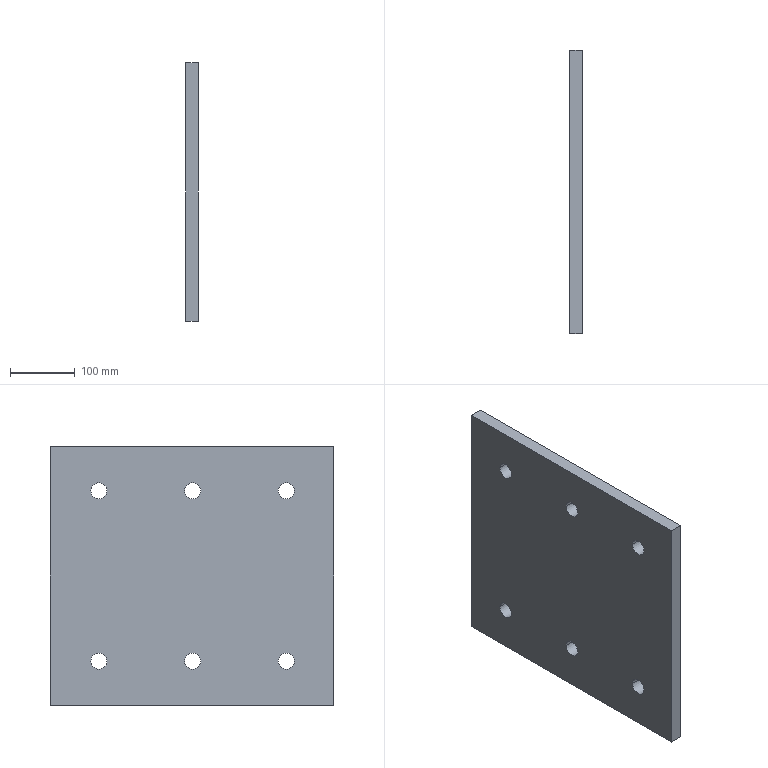Component | SolidWorks | ConnectingPlate-1 | 1 solid | 18 faces | box 20 x 438 x 400 mm | volume 3445095 mm3 | cylinder 12 | plane 6 | commonest cylinder face diameters 25 x12 | material Plain Carbon Steel
STEP:
#1=COLOUR_RGB('',0.7922,0.8196,0.9333);
#2=FILL_AREA_STYLE_COLOUR('',#1);
#3=FILL_AREA_STYLE('',(#2));
#4=SURFACE_STYLE_FILL_AREA(#3);
#5=SURFACE_SIDE_STYLE('',(#4));
#6=SURFACE_STYLE_USAGE(.BOTH.,#5);
#7=PRESENTATION_STYLE_ASSIGNMENT((#6));
#8=CARTESIAN_POINT('',(654.919,112.492,67.853));
#9=VERTEX_POINT('',#8);
#10=CARTESIAN_POINT('',(654.919,111.508,67.853));
#11=VERTEX_POINT('',#10);
#12=CARTESIAN_POINT('',(654.919,112.,67.853));
#13=DIRECTION('',(1.,-0.,-0.));
#14=DIRECTION('',(0.,1.,0.));
#15=AXIS2_PLACEMENT_3D('',#12,#13,#14);
#16=CIRCLE('',#15,0.4921);
#17=EDGE_CURVE('',#9,#11,#16,.T.);
#18=ORIENTED_EDGE('',*,*,#17,.F.);
#19=CARTESIAN_POINT('',(655.706,112.492,67.853));
#20=VERTEX_POINT('',#19);
#21=CARTESIAN_POINT('',(654.919,112.492,67.853));
#22=DIRECTION('',(1.,-0.,-0.));
#23=VECTOR('',#22,39.37);
#24=LINE('',#21,#23);
#25=EDGE_CURVE('',#9,#20,#24,.T.);
#26=ORIENTED_EDGE('',*,*,#25,.T.);
#27=CARTESIAN_POINT('',(655.706,111.508,67.853));
#28=VERTEX_POINT('',#27);
#29=CARTESIAN_POINT('',(655.706,112.,67.853));
#30=DIRECTION('',(1.,-0.,-0.));
#31=DIRECTION('',(0.,1.,0.));
#32=AXIS2_PLACEMENT_3D('',#29,#30,#31);
#33=CIRCLE('',#32,0.4921);
#34=EDGE_CURVE('',#20,#28,#33,.T.);
#35=ORIENTED_EDGE('',*,*,#34,.T.);
#36=CARTESIAN_POINT('',(654.919,111.508,67.853));
#37=DIRECTION('',(1.,-0.,-0.));
#38=VECTOR('',#37,39.37);
#39=LINE('',#36,#38);
#40=EDGE_CURVE('',#11,#28,#39,.T.);
#41=ORIENTED_EDGE('',*,*,#40,.F.);
#42=EDGE_LOOP('',(#18,#26,#35,#41));
#43=FACE_OUTER_BOUND('',#42,.T.);
#44=CARTESIAN_POINT('',(654.919,112.,67.853));
#45=DIRECTION('',(1.,-0.,-0.));
#46=DIRECTION('',(0.,-1.,0.));
#47=AXIS2_PLACEMENT_3D('',#44,#45,#46);
#48=CYLINDRICAL_SURFACE('',#47,0.4921);
#49=ADVANCED_FACE('',(#43),#48,.F.);
#50=CARTESIAN_POINT('',(654.919,106.784,67.853));
#51=VERTEX_POINT('',#50);
#52=CARTESIAN_POINT('',(654.919,105.799,67.853));
#53=VERTEX_POINT('',#52);
#54=CARTESIAN_POINT('',(654.919,106.291,67.853));
#55=DIRECTION('',(1.,-0.,-0.));
#56=DIRECTION('',(0.,1.,0.));
#57=AXIS2_PLACEMENT_3D('',#54,#55,#56);
#58=CIRCLE('',#57,0.4921);
#59=EDGE_CURVE('',#51,#53,#58,.T.);
#60=ORIENTED_EDGE('',*,*,#59,.F.);
#61=CARTESIAN_POINT('',(655.706,106.784,67.853));
#62=VERTEX_POINT('',#61);
#63=CARTESIAN_POINT('',(654.919,106.784,67.853));
#64=DIRECTION('',(1.,-0.,-0.));
#65=VECTOR('',#64,39.37);
#66=LINE('',#63,#65);
#67=EDGE_CURVE('',#51,#62,#66,.T.);
#68=ORIENTED_EDGE('',*,*,#67,.T.);
#69=CARTESIAN_POINT('',(655.706,105.799,67.853));
#70=VERTEX_POINT('',#69);
#71=CARTESIAN_POINT('',(655.706,106.291,67.853));
#72=DIRECTION('',(1.,-0.,-0.));
#73=DIRECTION('',(0.,1.,0.));
#74=AXIS2_PLACEMENT_3D('',#71,#72,#73);
#75=CIRCLE('',#74,0.4921);
#76=EDGE_CURVE('',#62,#70,#75,.T.);
#77=ORIENTED_EDGE('',*,*,#76,.T.);
#78=CARTESIAN_POINT('',(654.919,105.799,67.853));
#79=DIRECTION('',(1.,-0.,-0.));
#80=VECTOR('',#79,39.37);
#81=LINE('',#78,#80);
#82=EDGE_CURVE('',#53,#70,#81,.T.);
#83=ORIENTED_EDGE('',*,*,#82,.F.);
#84=EDGE_LOOP('',(#60,#68,#77,#83));
#85=FACE_OUTER_BOUND('',#84,.T.);
#86=CARTESIAN_POINT('',(654.919,106.291,67.853));
#87=DIRECTION('',(1.,-0.,-0.));
#88=DIRECTION('',(0.,-1.,0.));
#89=AXIS2_PLACEMENT_3D('',#86,#87,#88);
#90=CYLINDRICAL_SURFACE('',#89,0.4921);
#91=ADVANCED_FACE('',(#85),#90,.F.);
#92=CARTESIAN_POINT('',(654.919,101.075,67.853));
#93=VERTEX_POINT('',#92);
#94=CARTESIAN_POINT('',(654.919,100.091,67.853));
#95=VERTEX_POINT('',#94);
#96=CARTESIAN_POINT('',(654.919,100.583,67.853));
#97=DIRECTION('',(1.,-0.,-0.));
#98=DIRECTION('',(0.,1.,0.));
#99=AXIS2_PLACEMENT_3D('',#96,#97,#98);
#100=CIRCLE('',#99,0.4921);
#101=EDGE_CURVE('',#93,#95,#100,.T.);
#102=ORIENTED_EDGE('',*,*,#101,.F.);
#103=CARTESIAN_POINT('',(655.706,101.075,67.853));
#104=VERTEX_POINT('',#103);
#105=CARTESIAN_POINT('',(654.919,101.075,67.853));
#106=DIRECTION('',(1.,-0.,-0.));
#107=VECTOR('',#106,39.37);
#108=LINE('',#105,#107);
#109=EDGE_CURVE('',#93,#104,#108,.T.);
#110=ORIENTED_EDGE('',*,*,#109,.T.);
#111=CARTESIAN_POINT('',(655.706,100.091,67.853));
#112=VERTEX_POINT('',#111);
#113=CARTESIAN_POINT('',(655.706,100.583,67.853));
#114=DIRECTION('',(1.,-0.,-0.));
#115=DIRECTION('',(0.,1.,0.));
#116=AXIS2_PLACEMENT_3D('',#113,#114,#115);
#117=CIRCLE('',#116,0.4921);
#118=EDGE_CURVE('',#104,#112,#117,.T.);
#119=ORIENTED_EDGE('',*,*,#118,.T.);
#120=CARTESIAN_POINT('',(654.919,100.091,67.853));
#121=DIRECTION('',(1.,-0.,-0.));
#122=VECTOR('',#121,39.37);
#123=LINE('',#120,#122);
#124=EDGE_CURVE('',#95,#112,#123,.T.);
#125=ORIENTED_EDGE('',*,*,#124,.F.);
#126=EDGE_LOOP('',(#102,#110,#119,#125));
#127=FACE_OUTER_BOUND('',#126,.T.);
#128=CARTESIAN_POINT('',(654.919,100.583,67.853));
#129=DIRECTION('',(1.,-0.,-0.));
#130=DIRECTION('',(0.,-1.,0.));
#131=AXIS2_PLACEMENT_3D('',#128,#129,#130);
#132=CYLINDRICAL_SURFACE('',#131,0.4921);
#133=ADVANCED_FACE('',(#127),#132,.F.);
#134=CARTESIAN_POINT('',(654.919,101.075,78.232));
#135=VERTEX_POINT('',#134);
#136=CARTESIAN_POINT('',(654.919,100.091,78.232));
#137=VERTEX_POINT('',#136);
#138=CARTESIAN_POINT('',(654.919,100.583,78.232));
#139=DIRECTION('',(1.,-0.,-0.));
#140=DIRECTION('',(0.,-1.,0.));
#141=AXIS2_PLACEMENT_3D('',#138,#139,#140);
#142=CIRCLE('',#141,0.4921);
#143=EDGE_CURVE('',#135,#137,#142,.T.);
#144=ORIENTED_EDGE('',*,*,#143,.F.);
#145=CARTESIAN_POINT('',(655.706,101.075,78.232));
#146=VERTEX_POINT('',#145);
#147=CARTESIAN_POINT('',(654.919,101.075,78.232));
#148=DIRECTION('',(1.,-0.,-0.));
#149=VECTOR('',#148,39.37);
#150=LINE('',#147,#149);
#151=EDGE_CURVE('',#135,#146,#150,.T.);
#152=ORIENTED_EDGE('',*,*,#151,.T.);
#153=CARTESIAN_POINT('',(655.706,100.091,78.232));
#154=VERTEX_POINT('',#153);
#155=CARTESIAN_POINT('',(655.706,100.583,78.232));
#156=DIRECTION('',(1.,-0.,-0.));
#157=DIRECTION('',(0.,-1.,0.));
#158=AXIS2_PLACEMENT_3D('',#155,#156,#157);
#159=CIRCLE('',#158,0.4921);
#160=EDGE_CURVE('',#146,#154,#159,.T.);
#161=ORIENTED_EDGE('',*,*,#160,.T.);
#162=CARTESIAN_POINT('',(654.919,100.091,78.232));
#163=DIRECTION('',(1.,-0.,-0.));
#164=VECTOR('',#163,39.37);
#165=LINE('',#162,#164);
#166=EDGE_CURVE('',#137,#154,#165,.T.);
#167=ORIENTED_EDGE('',*,*,#166,.F.);
#168=EDGE_LOOP('',(#144,#152,#161,#167));
#169=FACE_OUTER_BOUND('',#168,.T.);
#170=CARTESIAN_POINT('',(654.919,100.583,78.232));
#171=DIRECTION('',(1.,-0.,-0.));
#172=DIRECTION('',(0.,-1.,0.));
#173=AXIS2_PLACEMENT_3D('',#170,#171,#172);
#174=CYLINDRICAL_SURFACE('',#173,0.4921);
#175=ADVANCED_FACE('',(#169),#174,.F.);
#176=CARTESIAN_POINT('',(654.919,106.784,78.232));
#177=VERTEX_POINT('',#176);
#178=CARTESIAN_POINT('',(654.919,105.799,78.232));
#179=VERTEX_POINT('',#178);
#180=CARTESIAN_POINT('',(654.919,106.291,78.232));
#181=DIRECTION('',(1.,-0.,-0.));
#182=DIRECTION('',(0.,-1.,0.));
#183=AXIS2_PLACEMENT_3D('',#180,#181,#182);
#184=CIRCLE('',#183,0.4921);
#185=EDGE_CURVE('',#177,#179,#184,.T.);
#186=ORIENTED_EDGE('',*,*,#185,.F.);
#187=CARTESIAN_POINT('',(655.706,106.784,78.232));
#188=VERTEX_POINT('',#187);
#189=CARTESIAN_POINT('',(654.919,106.784,78.232));
#190=DIRECTION('',(1.,-0.,-0.));
#191=VECTOR('',#190,39.37);
#192=LINE('',#189,#191);
#193=EDGE_CURVE('',#177,#188,#192,.T.);
#194=ORIENTED_EDGE('',*,*,#193,.T.);
#195=CARTESIAN_POINT('',(655.706,105.799,78.232));
#196=VERTEX_POINT('',#195);
#197=CARTESIAN_POINT('',(655.706,106.291,78.232));
#198=DIRECTION('',(1.,-0.,-0.));
#199=DIRECTION('',(0.,-1.,0.));
#200=AXIS2_PLACEMENT_3D('',#197,#198,#199);
#201=CIRCLE('',#200,0.4921);
#202=EDGE_CURVE('',#188,#196,#201,.T.);
#203=ORIENTED_EDGE('',*,*,#202,.T.);
#204=CARTESIAN_POINT('',(654.919,105.799,78.232));
#205=DIRECTION('',(1.,-0.,-0.));
#206=VECTOR('',#205,39.37);
#207=LINE('',#204,#206);
#208=EDGE_CURVE('',#179,#196,#207,.T.);
#209=ORIENTED_EDGE('',*,*,#208,.F.);
#210=EDGE_LOOP('',(#186,#194,#203,#209));
#211=FACE_OUTER_BOUND('',#210,.T.);
#212=CARTESIAN_POINT('',(654.919,106.291,78.232));
#213=DIRECTION('',(1.,-0.,-0.));
#214=DIRECTION('',(0.,-1.,0.));
#215=AXIS2_PLACEMENT_3D('',#212,#213,#214);
#216=CYLINDRICAL_SURFACE('',#215,0.4921);
#217=ADVANCED_FACE('',(#211),#216,.F.);
#218=CARTESIAN_POINT('',(654.919,112.492,78.232));
#219=VERTEX_POINT('',#218);
#220=CARTESIAN_POINT('',(654.919,111.508,78.232));
#221=VERTEX_POINT('',#220);
#222=CARTESIAN_POINT('',(654.919,112.,78.232));
#223=DIRECTION('',(1.,-0.,-0.));
#224=DIRECTION('',(0.,-1.,0.));
#225=AXIS2_PLACEMENT_3D('',#222,#223,#224);
#226=CIRCLE('',#225,0.4921);
#227=EDGE_CURVE('',#219,#221,#226,.T.);
#228=ORIENTED_EDGE('',*,*,#227,.F.);
#229=CARTESIAN_POINT('',(655.706,112.492,78.232));
#230=VERTEX_POINT('',#229);
#231=CARTESIAN_POINT('',(654.919,112.492,78.232));
#232=DIRECTION('',(1.,-0.,-0.));
#233=VECTOR('',#232,39.37);
#234=LINE('',#231,#233);
#235=EDGE_CURVE('',#219,#230,#234,.T.);
#236=ORIENTED_EDGE('',*,*,#235,.T.);
#237=CARTESIAN_POINT('',(655.706,111.508,78.232));
#238=VERTEX_POINT('',#237);
#239=CARTESIAN_POINT('',(655.706,112.,78.232));
#240=DIRECTION('',(1.,-0.,-0.));
#241=DIRECTION('',(0.,-1.,0.));
#242=AXIS2_PLACEMENT_3D('',#239,#240,#241);
#243=CIRCLE('',#242,0.4921);
#244=EDGE_CURVE('',#230,#238,#243,.T.);
#245=ORIENTED_EDGE('',*,*,#244,.T.);
#246=CARTESIAN_POINT('',(654.919,111.508,78.232));
#247=DIRECTION('',(1.,-0.,-0.));
#248=VECTOR('',#247,39.37);
#249=LINE('',#246,#248);
#250=EDGE_CURVE('',#221,#238,#249,.T.);
#251=ORIENTED_EDGE('',*,*,#250,.F.);
#252=EDGE_LOOP('',(#228,#236,#245,#251));
#253=FACE_OUTER_BOUND('',#252,.T.);
#254=CARTESIAN_POINT('',(654.919,112.,78.232));
#255=DIRECTION('',(1.,-0.,-0.));
#256=DIRECTION('',(0.,-1.,0.));
#257=AXIS2_PLACEMENT_3D('',#254,#255,#256);
#258=CYLINDRICAL_SURFACE('',#257,0.4921);
#259=ADVANCED_FACE('',(#253),#258,.F.);
#260=CARTESIAN_POINT('',(654.919,97.709,65.169));
#261=VERTEX_POINT('',#260);
#262=CARTESIAN_POINT('',(655.706,97.709,65.169));
#263=VERTEX_POINT('',#262);
#264=CARTESIAN_POINT('',(654.919,97.709,65.169));
#265=DIRECTION('',(1.,-0.,-0.));
#266=VECTOR('',#265,39.37);
#267=LINE('',#264,#266);
#268=EDGE_CURVE('',#261,#263,#267,.T.);
#269=ORIENTED_EDGE('',*,*,#268,.F.);
#270=CARTESIAN_POINT('',(654.919,114.953,65.169));
#271=VERTEX_POINT('',#270);
#272=CARTESIAN_POINT('',(654.919,114.953,65.169));
#273=DIRECTION('',(0.,1.,0.));
#274=VECTOR('',#273,39.37);
#275=LINE('',#272,#274);
#276=EDGE_CURVE('',#261,#271,#275,.T.);
#277=ORIENTED_EDGE('',*,*,#276,.T.);
#278=CARTESIAN_POINT('',(655.706,114.953,65.169));
#279=VERTEX_POINT('',#278);
#280=CARTESIAN_POINT('',(654.919,114.953,65.169));
#281=DIRECTION('',(1.,-0.,-0.));
#282=VECTOR('',#281,39.37);
#283=LINE('',#280,#282);
#284=EDGE_CURVE('',#271,#279,#283,.T.);
#285=ORIENTED_EDGE('',*,*,#284,.T.);
#286=CARTESIAN_POINT('',(655.706,114.953,65.169));
#287=DIRECTION('',(0.,1.,0.));
#288=VECTOR('',#287,39.37);
#289=LINE('',#286,#288);
#290=EDGE_CURVE('',#263,#279,#289,.T.);
#291=ORIENTED_EDGE('',*,*,#290,.F.);
#292=EDGE_LOOP('',(#269,#277,#285,#291));
#293=FACE_OUTER_BOUND('',#292,.T.);
#294=CARTESIAN_POINT('',(654.919,114.953,65.169));
#295=DIRECTION('',(-0.,0.,-1.));
#296=DIRECTION('',(0.,1.,0.));
#297=AXIS2_PLACEMENT_3D('',#294,#295,#296);
#298=PLANE('',#297);
#299=ADVANCED_FACE('',(#293),#298,.T.);
#300=CARTESIAN_POINT('',(655.706,97.709,80.917));
#301=VERTEX_POINT('',#300);
#302=CARTESIAN_POINT('',(654.919,97.709,80.917));
#303=VERTEX_POINT('',#302);
#304=CARTESIAN_POINT('',(654.919,97.709,80.917));
#305=DIRECTION('',(-1.,0.,0.));
#306=VECTOR('',#305,39.37);
#307=LINE('',#304,#306);
#308=EDGE_CURVE('',#301,#303,#307,.T.);
#309=ORIENTED_EDGE('',*,*,#308,.F.);
#310=CARTESIAN_POINT('',(655.706,114.953,80.917));
#311=VERTEX_POINT('',#310);
#312=CARTESIAN_POINT('',(655.706,114.953,80.917));
#313=DIRECTION('',(-0.,-1.,-0.));
#314=VECTOR('',#313,39.37);
#315=LINE('',#312,#314);
#316=EDGE_CURVE('',#311,#301,#315,.T.);
#317=ORIENTED_EDGE('',*,*,#316,.F.);
#318=CARTESIAN_POINT('',(654.919,114.953,80.917));
#319=VERTEX_POINT('',#318);
#320=CARTESIAN_POINT('',(654.919,114.953,80.917));
#321=DIRECTION('',(1.,-0.,-0.));
#322=VECTOR('',#321,39.37);
#323=LINE('',#320,#322);
#324=EDGE_CURVE('',#319,#311,#323,.T.);
#325=ORIENTED_EDGE('',*,*,#324,.F.);
#326=CARTESIAN_POINT('',(654.919,114.953,80.917));
#327=DIRECTION('',(-0.,-1.,-0.));
#328=VECTOR('',#327,39.37);
#329=LINE('',#326,#328);
#330=EDGE_CURVE('',#319,#303,#329,.T.);
#331=ORIENTED_EDGE('',*,*,#330,.T.);
#332=EDGE_LOOP('',(#309,#317,#325,#331));
#333=FACE_OUTER_BOUND('',#332,.T.);
#334=CARTESIAN_POINT('',(654.919,114.953,80.917));
#335=DIRECTION('',(0.,-0.,1.));
#336=DIRECTION('',(-0.,-1.,-0.));
#337=AXIS2_PLACEMENT_3D('',#334,#335,#336);
#338=PLANE('',#337);
#339=ADVANCED_FACE('',(#333),#338,.T.);
#340=CARTESIAN_POINT('',(655.706,114.953,80.917));
#341=DIRECTION('',(0.,0.,1.));
#342=VECTOR('',#341,39.37);
#343=LINE('',#340,#342);
#344=EDGE_CURVE('',#279,#311,#343,.T.);
#345=ORIENTED_EDGE('',*,*,#344,.F.);
#346=ORIENTED_EDGE('',*,*,#284,.F.);
#347=CARTESIAN_POINT('',(654.919,114.953,80.917));
#348=DIRECTION('',(0.,0.,1.));
#349=VECTOR('',#348,39.37);
#350=LINE('',#347,#349);
#351=EDGE_CURVE('',#271,#319,#350,.T.);
#352=ORIENTED_EDGE('',*,*,#351,.T.);
#353=ORIENTED_EDGE('',*,*,#324,.T.);
#354=EDGE_LOOP('',(#345,#346,#352,#353));
#355=FACE_OUTER_BOUND('',#354,.T.);
#356=CARTESIAN_POINT('',(654.919,114.953,80.917));
#357=DIRECTION('',(0.,1.,-0.));
#358=DIRECTION('',(0.,0.,1.));
#359=AXIS2_PLACEMENT_3D('',#356,#357,#358);
#360=PLANE('',#359);
#361=ADVANCED_FACE('',(#355),#360,.T.);
#362=CARTESIAN_POINT('',(654.919,112.,67.853));
#363=DIRECTION('',(1.,-0.,-0.));
#364=DIRECTION('',(0.,1.,0.));
#365=AXIS2_PLACEMENT_3D('',#362,#363,#364);
#366=CIRCLE('',#365,0.4921);
#367=EDGE_CURVE('',#11,#9,#366,.T.);
#368=ORIENTED_EDGE('',*,*,#367,.T.);
#369=ORIENTED_EDGE('',*,*,#17,.T.);
#370=EDGE_LOOP('',(#368,#369));
#371=FACE_BOUND('',#370,.T.);
#372=CARTESIAN_POINT('',(654.919,106.291,67.853));
#373=DIRECTION('',(1.,-0.,-0.));
#374=DIRECTION('',(0.,1.,0.));
#375=AXIS2_PLACEMENT_3D('',#372,#373,#374);
#376=CIRCLE('',#375,0.4921);
#377=EDGE_CURVE('',#53,#51,#376,.T.);
#378=ORIENTED_EDGE('',*,*,#377,.T.);
#379=ORIENTED_EDGE('',*,*,#59,.T.);
#380=EDGE_LOOP('',(#378,#379));
#381=FACE_BOUND('',#380,.T.);
#382=CARTESIAN_POINT('',(654.919,100.583,67.853));
#383=DIRECTION('',(1.,-0.,-0.));
#384=DIRECTION('',(0.,1.,0.));
#385=AXIS2_PLACEMENT_3D('',#382,#383,#384);
#386=CIRCLE('',#385,0.4921);
#387=EDGE_CURVE('',#95,#93,#386,.T.);
#388=ORIENTED_EDGE('',*,*,#387,.T.);
#389=ORIENTED_EDGE('',*,*,#101,.T.);
#390=EDGE_LOOP('',(#388,#389));
#391=FACE_BOUND('',#390,.T.);
#392=CARTESIAN_POINT('',(654.919,100.583,78.232));
#393=DIRECTION('',(1.,-0.,-0.));
#394=DIRECTION('',(0.,-1.,0.));
#395=AXIS2_PLACEMENT_3D('',#392,#393,#394);
#396=CIRCLE('',#395,0.4921);
#397=EDGE_CURVE('',#137,#135,#396,.T.);
#398=ORIENTED_EDGE('',*,*,#397,.T.);
#399=ORIENTED_EDGE('',*,*,#143,.T.);
#400=EDGE_LOOP('',(#398,#399));
#401=FACE_BOUND('',#400,.T.);
#402=CARTESIAN_POINT('',(654.919,106.291,78.232));
#403=DIRECTION('',(1.,-0.,-0.));
#404=DIRECTION('',(0.,-1.,0.));
#405=AXIS2_PLACEMENT_3D('',#402,#403,#404);
#406=CIRCLE('',#405,0.4921);
#407=EDGE_CURVE('',#179,#177,#406,.T.);
#408=ORIENTED_EDGE('',*,*,#407,.T.);
#409=ORIENTED_EDGE('',*,*,#185,.T.);
#410=EDGE_LOOP('',(#408,#409));
#411=FACE_BOUND('',#410,.T.);
#412=CARTESIAN_POINT('',(654.919,112.,78.232));
#413=DIRECTION('',(1.,-0.,-0.));
#414=DIRECTION('',(0.,-1.,0.));
#415=AXIS2_PLACEMENT_3D('',#412,#413,#414);
#416=CIRCLE('',#415,0.4921);
#417=EDGE_CURVE('',#221,#219,#416,.T.);
#418=ORIENTED_EDGE('',*,*,#417,.T.);
#419=ORIENTED_EDGE('',*,*,#227,.T.);
#420=EDGE_LOOP('',(#418,#419));
#421=FACE_BOUND('',#420,.T.);
#422=ORIENTED_EDGE('',*,*,#276,.F.);
#423=CARTESIAN_POINT('',(654.919,97.709,81.311));
#424=DIRECTION('',(0.,0.,1.));
#425=VECTOR('',#424,39.37);
#426=LINE('',#423,#425);
#427=EDGE_CURVE('',#261,#303,#426,.T.);
#428=ORIENTED_EDGE('',*,*,#427,.T.);
#429=ORIENTED_EDGE('',*,*,#330,.F.);
#430=ORIENTED_EDGE('',*,*,#351,.F.);
#431=EDGE_LOOP('',(#422,#428,#429,#430));
#432=FACE_OUTER_BOUND('',#431,.T.);
#433=CARTESIAN_POINT('',(654.919,106.291,73.043));
#434=DIRECTION('',(1.,-0.,-0.));
#435=DIRECTION('',(-0.,-1.,0.));
#436=AXIS2_PLACEMENT_3D('',#433,#434,#435);
#437=PLANE('',#436);
#438=ADVANCED_FACE('',(#371,#381,#391,#401,#411,#421,#432),#437,.F.);
#439=CARTESIAN_POINT('',(655.706,97.709,73.043));
#440=DIRECTION('',(0.,0.,1.));
#441=VECTOR('',#440,39.37);
#442=LINE('',#439,#441);
#443=EDGE_CURVE('',#263,#301,#442,.T.);
#444=ORIENTED_EDGE('',*,*,#443,.F.);
#445=ORIENTED_EDGE('',*,*,#290,.T.);
#446=ORIENTED_EDGE('',*,*,#344,.T.);
#447=ORIENTED_EDGE('',*,*,#316,.T.);
#448=EDGE_LOOP('',(#444,#445,#446,#447));
#449=FACE_OUTER_BOUND('',#448,.T.);
#450=CARTESIAN_POINT('',(655.706,112.,67.853));
#451=DIRECTION('',(1.,-0.,-0.));
#452=DIRECTION('',(0.,1.,0.));
#453=AXIS2_PLACEMENT_3D('',#450,#451,#452);
#454=CIRCLE('',#453,0.4921);
#455=EDGE_CURVE('',#28,#20,#454,.T.);
#456=ORIENTED_EDGE('',*,*,#455,.F.);
#457=ORIENTED_EDGE('',*,*,#34,.F.);
#458=EDGE_LOOP('',(#456,#457));
#459=FACE_BOUND('',#458,.T.);
#460=CARTESIAN_POINT('',(655.706,106.291,67.853));
#461=DIRECTION('',(1.,-0.,-0.));
#462=DIRECTION('',(0.,1.,0.));
#463=AXIS2_PLACEMENT_3D('',#460,#461,#462);
#464=CIRCLE('',#463,0.4921);
#465=EDGE_CURVE('',#70,#62,#464,.T.);
#466=ORIENTED_EDGE('',*,*,#465,.F.);
#467=ORIENTED_EDGE('',*,*,#76,.F.);
#468=EDGE_LOOP('',(#466,#467));
#469=FACE_BOUND('',#468,.T.);
#470=CARTESIAN_POINT('',(655.706,100.583,67.853));
#471=DIRECTION('',(1.,-0.,-0.));
#472=DIRECTION('',(0.,1.,0.));
#473=AXIS2_PLACEMENT_3D('',#470,#471,#472);
#474=CIRCLE('',#473,0.4921);
#475=EDGE_CURVE('',#112,#104,#474,.T.);
#476=ORIENTED_EDGE('',*,*,#475,.F.);
#477=ORIENTED_EDGE('',*,*,#118,.F.);
#478=EDGE_LOOP('',(#476,#477));
#479=FACE_BOUND('',#478,.T.);
#480=CARTESIAN_POINT('',(655.706,100.583,78.232));
#481=DIRECTION('',(1.,-0.,-0.));
#482=DIRECTION('',(0.,-1.,0.));
#483=AXIS2_PLACEMENT_3D('',#480,#481,#482);
#484=CIRCLE('',#483,0.4921);
#485=EDGE_CURVE('',#154,#146,#484,.T.);
#486=ORIENTED_EDGE('',*,*,#485,.F.);
#487=ORIENTED_EDGE('',*,*,#160,.F.);
#488=EDGE_LOOP('',(#486,#487));
#489=FACE_BOUND('',#488,.T.);
#490=CARTESIAN_POINT('',(655.706,106.291,78.232));
#491=DIRECTION('',(1.,-0.,-0.));
#492=DIRECTION('',(0.,-1.,0.));
#493=AXIS2_PLACEMENT_3D('',#490,#491,#492);
#494=CIRCLE('',#493,0.4921);
#495=EDGE_CURVE('',#196,#188,#494,.T.);
#496=ORIENTED_EDGE('',*,*,#495,.F.);
#497=ORIENTED_EDGE('',*,*,#202,.F.);
#498=EDGE_LOOP('',(#496,#497));
#499=FACE_BOUND('',#498,.T.);
#500=CARTESIAN_POINT('',(655.706,112.,78.232));
#501=DIRECTION('',(1.,-0.,-0.));
#502=DIRECTION('',(0.,-1.,0.));
#503=AXIS2_PLACEMENT_3D('',#500,#501,#502);
#504=CIRCLE('',#503,0.4921);
#505=EDGE_CURVE('',#238,#230,#504,.T.);
#506=ORIENTED_EDGE('',*,*,#505,.F.);
#507=ORIENTED_EDGE('',*,*,#244,.F.);
#508=EDGE_LOOP('',(#506,#507));
#509=FACE_BOUND('',#508,.T.);
#510=CARTESIAN_POINT('',(655.706,106.291,73.043));
#511=DIRECTION('',(1.,-0.,-0.));
#512=DIRECTION('',(-0.,-1.,0.));
#513=AXIS2_PLACEMENT_3D('',#510,#511,#512);
#514=PLANE('',#513);
#515=ADVANCED_FACE('',(#449,#459,#469,#479,#489,#499,#509),#514,.T.);
#516=ORIENTED_EDGE('',*,*,#235,.F.);
#517=ORIENTED_EDGE('',*,*,#417,.F.);
#518=ORIENTED_EDGE('',*,*,#250,.T.);
#519=ORIENTED_EDGE('',*,*,#505,.T.);
#520=EDGE_LOOP('',(#516,#517,#518,#519));
#521=FACE_OUTER_BOUND('',#520,.T.);
#522=CARTESIAN_POINT('',(654.919,112.,78.232));
#523=DIRECTION('',(1.,-0.,-0.));
#524=DIRECTION('',(0.,-1.,0.));
#525=AXIS2_PLACEMENT_3D('',#522,#523,#524);
#526=CYLINDRICAL_SURFACE('',#525,0.4921);
#527=ADVANCED_FACE('',(#521),#526,.F.);
#528=ORIENTED_EDGE('',*,*,#193,.F.);
#529=ORIENTED_EDGE('',*,*,#407,.F.);
#530=ORIENTED_EDGE('',*,*,#208,.T.);
#531=ORIENTED_EDGE('',*,*,#495,.T.);
#532=EDGE_LOOP('',(#528,#529,#530,#531));
#533=FACE_OUTER_BOUND('',#532,.T.);
#534=CARTESIAN_POINT('',(654.919,106.291,78.232));
#535=DIRECTION('',(1.,-0.,-0.));
#536=DIRECTION('',(0.,-1.,0.));
#537=AXIS2_PLACEMENT_3D('',#534,#535,#536);
#538=CYLINDRICAL_SURFACE('',#537,0.4921);
#539=ADVANCED_FACE('',(#533),#538,.F.);
#540=ORIENTED_EDGE('',*,*,#151,.F.);
#541=ORIENTED_EDGE('',*,*,#397,.F.);
#542=ORIENTED_EDGE('',*,*,#166,.T.);
#543=ORIENTED_EDGE('',*,*,#485,.T.);
#544=EDGE_LOOP('',(#540,#541,#542,#543));
#545=FACE_OUTER_BOUND('',#544,.T.);
#546=CARTESIAN_POINT('',(654.919,100.583,78.232));
#547=DIRECTION('',(1.,-0.,-0.));
#548=DIRECTION('',(0.,-1.,0.));
#549=AXIS2_PLACEMENT_3D('',#546,#547,#548);
#550=CYLINDRICAL_SURFACE('',#549,0.4921);
#551=ADVANCED_FACE('',(#545),#550,.F.);
#552=ORIENTED_EDGE('',*,*,#109,.F.);
#553=ORIENTED_EDGE('',*,*,#387,.F.);
#554=ORIENTED_EDGE('',*,*,#124,.T.);
#555=ORIENTED_EDGE('',*,*,#475,.T.);
#556=EDGE_LOOP('',(#552,#553,#554,#555));
#557=FACE_OUTER_BOUND('',#556,.T.);
#558=CARTESIAN_POINT('',(654.919,100.583,67.853));
#559=DIRECTION('',(1.,-0.,-0.));
#560=DIRECTION('',(0.,-1.,0.));
#561=AXIS2_PLACEMENT_3D('',#558,#559,#560);
#562=CYLINDRICAL_SURFACE('',#561,0.4921);
#563=ADVANCED_FACE('',(#557),#562,.F.);
#564=ORIENTED_EDGE('',*,*,#67,.F.);
#565=ORIENTED_EDGE('',*,*,#377,.F.);
#566=ORIENTED_EDGE('',*,*,#82,.T.);
#567=ORIENTED_EDGE('',*,*,#465,.T.);
#568=EDGE_LOOP('',(#564,#565,#566,#567));
#569=FACE_OUTER_BOUND('',#568,.T.);
#570=CARTESIAN_POINT('',(654.919,106.291,67.853));
#571=DIRECTION('',(1.,-0.,-0.));
#572=DIRECTION('',(0.,-1.,0.));
#573=AXIS2_PLACEMENT_3D('',#570,#571,#572);
#574=CYLINDRICAL_SURFACE('',#573,0.4921);
#575=ADVANCED_FACE('',(#569),#574,.F.);
#576=ORIENTED_EDGE('',*,*,#25,.F.);
#577=ORIENTED_EDGE('',*,*,#367,.F.);
#578=ORIENTED_EDGE('',*,*,#40,.T.);
#579=ORIENTED_EDGE('',*,*,#455,.T.);
#580=EDGE_LOOP('',(#576,#577,#578,#579));
#581=FACE_OUTER_BOUND('',#580,.T.);
#582=CARTESIAN_POINT('',(654.919,112.,67.853));
#583=DIRECTION('',(1.,-0.,-0.));
#584=DIRECTION('',(0.,-1.,0.));
#585=AXIS2_PLACEMENT_3D('',#582,#583,#584);
#586=CYLINDRICAL_SURFACE('',#585,0.4921);
#587=ADVANCED_FACE('',(#581),#586,.F.);
#588=ORIENTED_EDGE('',*,*,#268,.T.);
#589=ORIENTED_EDGE('',*,*,#443,.T.);
#590=ORIENTED_EDGE('',*,*,#308,.T.);
#591=ORIENTED_EDGE('',*,*,#427,.F.);
#592=EDGE_LOOP('',(#588,#589,#590,#591));
#593=FACE_OUTER_BOUND('',#592,.T.);
#594=CARTESIAN_POINT('',(654.919,97.709,81.311));
#595=DIRECTION('',(0.,1.,-0.));
#596=DIRECTION('',(0.,0.,1.));
#597=AXIS2_PLACEMENT_3D('',#594,#595,#596);
#598=PLANE('',#597);
#599=ADVANCED_FACE('',(#593),#598,.F.);
#600=CLOSED_SHELL('',(#49,#91,#133,#175,#217,#259,#299,#339,#361,#438,#515,#527,#539,#551,#563,#575,#587,#599));
#601=MANIFOLD_SOLID_BREP('',#600);
#602=STYLED_ITEM('',(#7),#601);
#603=PRESENTATION_LAYER_ASSIGNMENT('','',(#602));
#604=CARTESIAN_POINT('',(0.,0.,0.));
#605=DIRECTION('',(0.,0.,1.));
#606=DIRECTION('',(1.,0.,0.));
#607=AXIS2_PLACEMENT_3D('',#604,#605,#606);
#608=(LENGTH_UNIT()NAMED_UNIT(*)SI_UNIT($,.METRE.));
#609=LENGTH_MEASURE_WITH_UNIT(LENGTH_MEASURE(0.0254),#608);
#610=DIMENSIONAL_EXPONENTS(1.,0.,0.,0.,0.,0.,0.);
#611=(CONVERSION_BASED_UNIT('',#609)LENGTH_UNIT()NAMED_UNIT(#610));
#612=UNCERTAINTY_MEASURE_WITH_UNIT(LENGTH_MEASURE(0.00001),#611,'','');
#613=(NAMED_UNIT(*)PLANE_ANGLE_UNIT()SI_UNIT($,.RADIAN.));
#614=(NAMED_UNIT(*)SI_UNIT($,.STERADIAN.)SOLID_ANGLE_UNIT());
#615=(GEOMETRIC_REPRESENTATION_CONTEXT(3)GLOBAL_UNCERTAINTY_ASSIGNED_CONTEXT((#612))GLOBAL_UNIT_ASSIGNED_CONTEXT((#611,#613,#614))REPRESENTATION_CONTEXT('',''));
#616=ADVANCED_BREP_SHAPE_REPRESENTATION('',(#601,#607),#615);
#617=(LENGTH_UNIT()NAMED_UNIT(*)SI_UNIT($,.METRE.));
#618=LENGTH_MEASURE_WITH_UNIT(LENGTH_MEASURE(0.0254),#617);
#619=DIMENSIONAL_EXPONENTS(1.,0.,0.,0.,0.,0.,0.);
#620=(CONVERSION_BASED_UNIT('',#618)LENGTH_UNIT()NAMED_UNIT(#619));
#621=UNCERTAINTY_MEASURE_WITH_UNIT(LENGTH_MEASURE(0.00001),#620,'','');
#622=(NAMED_UNIT(*)PLANE_ANGLE_UNIT()SI_UNIT($,.RADIAN.));
#623=(NAMED_UNIT(*)SI_UNIT($,.STERADIAN.)SOLID_ANGLE_UNIT());
#624=(GEOMETRIC_REPRESENTATION_CONTEXT(3)GLOBAL_UNCERTAINTY_ASSIGNED_CONTEXT((#621))GLOBAL_UNIT_ASSIGNED_CONTEXT((#620,#622,#623))REPRESENTATION_CONTEXT('',''));
#625=MECHANICAL_DESIGN_GEOMETRIC_PRESENTATION_REPRESENTATION('',(#602),#624);